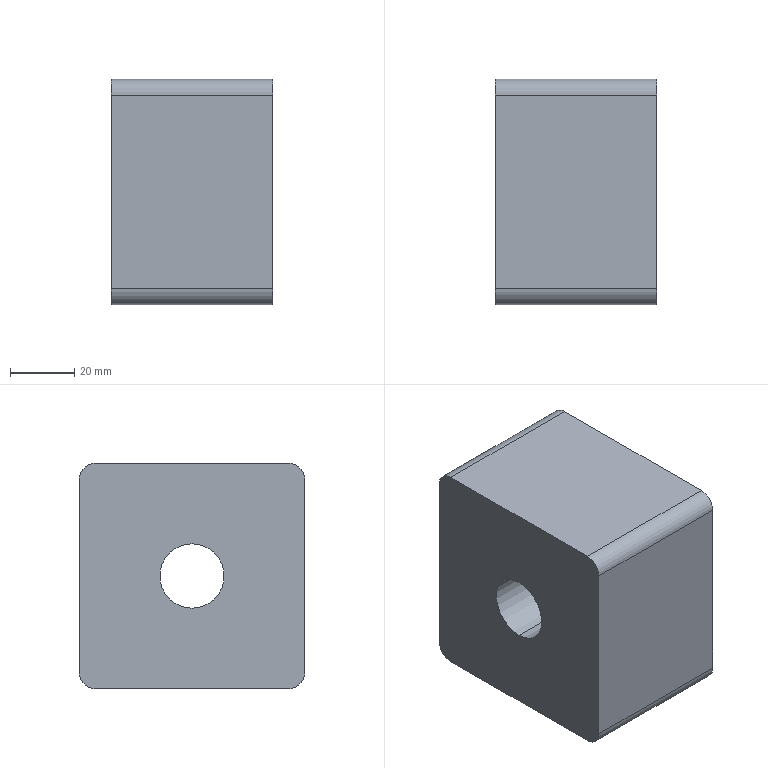Component | SolidWorks | ArmServoMotorAssembly-1_ArmServoMotor-1 | 1 solid | 12 faces | box 50 x 70 x 70 mm | volume 228219 mm3 | cylinder 6 | plane 6 | commonest cylinder face diameters 10 x4 20 x2
build123d program:
from build123d import *

# Parameters (mm, degrees)
SKETCH1_W           = 70
SKETCH1_H           = 70
BOSS_EXTRUDE1_DEPTH = 50
FILLET1_R           = 5
CUT_EXTRUDE1_REACH  = 72.356
SKETCH2_R           = 10


with BuildPart() as part:
    # Sketch1 → Boss-Extrude1 (new body)
    with BuildSketch(Plane.XY):
        Rectangle(SKETCH1_W, SKETCH1_H)
    extrude(amount=BOSS_EXTRUDE1_DEPTH)

    # Fillet1
    fillet1_edges = [part.edges().sort_by_distance(p)[0] for p in [
        (35, -35, 25),
        (-35, -35, 25),
        (-35, 35, 25),
        (35, 35, 25),
    ]]
    fillet(fillet1_edges, radius=FILLET1_R)

    # Sketch2 → Cut-Extrude1 (cut, up to next)
    with BuildSketch(Plane.XY.offset(50), mode=Mode.PRIVATE) as cut_extrude1_sk1:
        Circle(SKETCH2_R)
    cut_extrude1_tool1 = extrude(cut_extrude1_sk1.sketch, amount=-CUT_EXTRUDE1_REACH, mode=Mode.PRIVATE) & part.part
    add(cut_extrude1_tool1.solids().sort_by_distance((0, 0, 50))[0], mode=Mode.SUBTRACT)


solid = part.part

# Placed as in the assembly
solid = solid.moved(Location((-34.359, 70.663, 0), (0, 90, 0)))